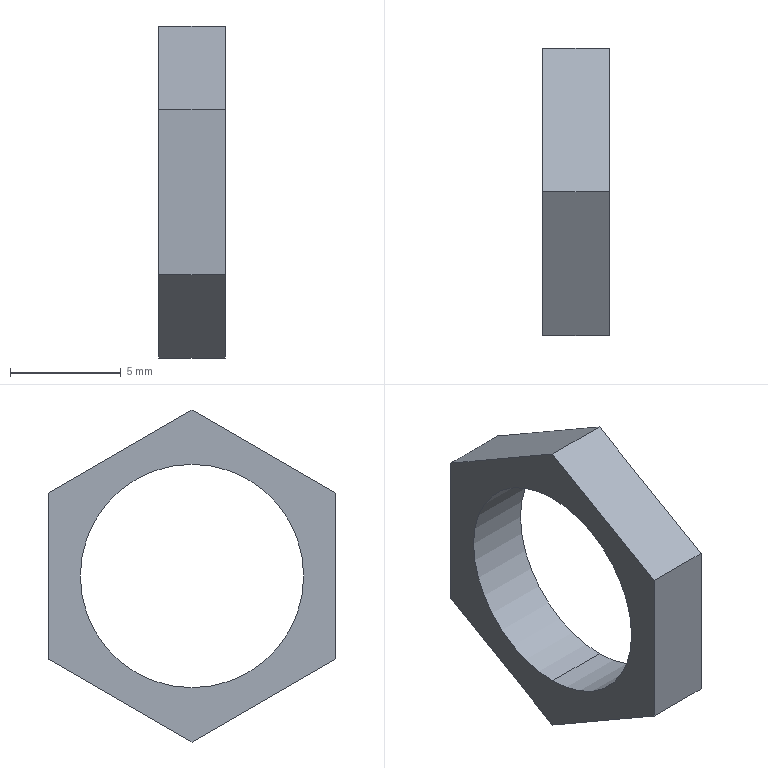Component | SolidWorks | GuideMechanism-1_SwingArm-1_AngleDisplacementSensorNut.1-1 | 1 solid | 10 faces | box 3 x 13 x 15.01 mm | volume 199 mm3 | plane 8 | cylinder 2 | commonest cylinder face diameters 10.1 x2
build123d program:
from build123d import *

# Parameters (mm, degrees)
BOSS_EXTRUDE1_DEPTH    = 3
M10X1_0_TAPPED_HOLE1_D = 10.1


with BuildPart() as part:
    # Sketch1 → Boss-Extrude1 (new body)
    with BuildSketch(Plane.XY):
        Polygon((7.506, 0), (3.753, 6.5), (-3.753, 6.5), (-7.506, 0), (-3.753, -6.5), (3.753, -6.5), align=None)
    extrude(amount=BOSS_EXTRUDE1_DEPTH)

    # M10x1.0 Tapped Hole1 (through all)
    with Locations(Plane(origin=(0, 0, 0), x_dir=(-1, 0, 0), z_dir=(0, 0, -1))):
        with Locations((0, 0)):
            Hole(M10X1_0_TAPPED_HOLE1_D / 2)


solid = part.part

# Placed as in the assembly
solid = solid.moved(Location((-615.272, -568.766, 1326.45), (0, 90, 0)))
STEP:
#1=CARTESIAN_POINT('',(-24.223,-22.392,52.024));
#2=VERTEX_POINT('',#1);
#3=CARTESIAN_POINT('',(-24.223,-22.392,52.421));
#4=VERTEX_POINT('',#3);
#5=CARTESIAN_POINT('',(-24.223,-22.392,52.222));
#6=DIRECTION('',(1.,-0.,0.));
#7=DIRECTION('',(0.,0.,1.));
#8=AXIS2_PLACEMENT_3D('',#5,#6,#7);
#9=CIRCLE('',#8,0.1988);
#10=EDGE_CURVE('',#2,#4,#9,.T.);
#11=ORIENTED_EDGE('',*,*,#10,.F.);
#12=CARTESIAN_POINT('',(-24.105,-22.392,52.024));
#13=VERTEX_POINT('',#12);
#14=CARTESIAN_POINT('',(-24.105,-22.392,52.024));
#15=DIRECTION('',(1.,-0.,0.));
#16=VECTOR('',#15,39.37);
#17=LINE('',#14,#16);
#18=EDGE_CURVE('',#2,#13,#17,.T.);
#19=ORIENTED_EDGE('',*,*,#18,.T.);
#20=CARTESIAN_POINT('',(-24.105,-22.392,52.421));
#21=VERTEX_POINT('',#20);
#22=CARTESIAN_POINT('',(-24.105,-22.392,52.222));
#23=DIRECTION('',(1.,-0.,0.));
#24=DIRECTION('',(0.,0.,1.));
#25=AXIS2_PLACEMENT_3D('',#22,#23,#24);
#26=CIRCLE('',#25,0.1988);
#27=EDGE_CURVE('',#13,#21,#26,.T.);
#28=ORIENTED_EDGE('',*,*,#27,.T.);
#29=CARTESIAN_POINT('',(-24.105,-22.392,52.421));
#30=DIRECTION('',(1.,-0.,0.));
#31=VECTOR('',#30,39.37);
#32=LINE('',#29,#31);
#33=EDGE_CURVE('',#4,#21,#32,.T.);
#34=ORIENTED_EDGE('',*,*,#33,.F.);
#35=EDGE_LOOP('',(#11,#19,#28,#34));
#36=FACE_OUTER_BOUND('',#35,.T.);
#37=CARTESIAN_POINT('',(-24.105,-22.392,52.222));
#38=DIRECTION('',(1.,-0.,0.));
#39=DIRECTION('',(0.,0.,1.));
#40=AXIS2_PLACEMENT_3D('',#37,#38,#39);
#41=CYLINDRICAL_SURFACE('',#40,0.1988);
#42=ADVANCED_FACE('',(#36),#41,.F.);
#43=CARTESIAN_POINT('',(-24.105,-22.136,52.075));
#44=VERTEX_POINT('',#43);
#45=CARTESIAN_POINT('',(-24.105,-22.392,51.927));
#46=VERTEX_POINT('',#45);
#47=CARTESIAN_POINT('',(-24.105,-22.136,52.075));
#48=DIRECTION('',(0.,-0.866,-0.5));
#49=VECTOR('',#48,39.37);
#50=LINE('',#47,#49);
#51=EDGE_CURVE('',#44,#46,#50,.T.);
#52=ORIENTED_EDGE('',*,*,#51,.T.);
#53=CARTESIAN_POINT('',(-24.223,-22.392,51.927));
#54=VERTEX_POINT('',#53);
#55=CARTESIAN_POINT('',(-24.223,-22.392,51.927));
#56=DIRECTION('',(1.,-0.,0.));
#57=VECTOR('',#56,39.37);
#58=LINE('',#55,#57);
#59=EDGE_CURVE('',#54,#46,#58,.T.);
#60=ORIENTED_EDGE('',*,*,#59,.F.);
#61=CARTESIAN_POINT('',(-24.223,-22.136,52.075));
#62=VERTEX_POINT('',#61);
#63=CARTESIAN_POINT('',(-24.223,-22.136,52.075));
#64=DIRECTION('',(0.,-0.866,-0.5));
#65=VECTOR('',#64,39.37);
#66=LINE('',#63,#65);
#67=EDGE_CURVE('',#62,#54,#66,.T.);
#68=ORIENTED_EDGE('',*,*,#67,.F.);
#69=CARTESIAN_POINT('',(-24.223,-22.136,52.075));
#70=DIRECTION('',(1.,-0.,0.));
#71=VECTOR('',#70,39.37);
#72=LINE('',#69,#71);
#73=EDGE_CURVE('',#62,#44,#72,.T.);
#74=ORIENTED_EDGE('',*,*,#73,.T.);
#75=EDGE_LOOP('',(#52,#60,#68,#74));
#76=FACE_OUTER_BOUND('',#75,.T.);
#77=CARTESIAN_POINT('',(-24.223,-22.136,52.075));
#78=DIRECTION('',(-0.,-0.5,0.866));
#79=DIRECTION('',(-0.,0.866,0.5));
#80=AXIS2_PLACEMENT_3D('',#77,#78,#79);
#81=PLANE('',#80);
#82=ADVANCED_FACE('',(#76),#81,.F.);
#83=CARTESIAN_POINT('',(-24.105,-22.648,52.075));
#84=VERTEX_POINT('',#83);
#85=CARTESIAN_POINT('',(-24.105,-22.392,51.927));
#86=DIRECTION('',(-0.,-0.866,0.5));
#87=VECTOR('',#86,39.37);
#88=LINE('',#85,#87);
#89=EDGE_CURVE('',#46,#84,#88,.T.);
#90=ORIENTED_EDGE('',*,*,#89,.T.);
#91=CARTESIAN_POINT('',(-24.223,-22.648,52.075));
#92=VERTEX_POINT('',#91);
#93=CARTESIAN_POINT('',(-24.223,-22.648,52.075));
#94=DIRECTION('',(1.,-0.,0.));
#95=VECTOR('',#94,39.37);
#96=LINE('',#93,#95);
#97=EDGE_CURVE('',#92,#84,#96,.T.);
#98=ORIENTED_EDGE('',*,*,#97,.F.);
#99=CARTESIAN_POINT('',(-24.223,-22.392,51.927));
#100=DIRECTION('',(-0.,-0.866,0.5));
#101=VECTOR('',#100,39.37);
#102=LINE('',#99,#101);
#103=EDGE_CURVE('',#54,#92,#102,.T.);
#104=ORIENTED_EDGE('',*,*,#103,.F.);
#105=ORIENTED_EDGE('',*,*,#59,.T.);
#106=EDGE_LOOP('',(#90,#98,#104,#105));
#107=FACE_OUTER_BOUND('',#106,.T.);
#108=CARTESIAN_POINT('',(-24.223,-22.392,51.927));
#109=DIRECTION('',(-0.,0.5,0.866));
#110=DIRECTION('',(0.,0.866,-0.5));
#111=AXIS2_PLACEMENT_3D('',#108,#109,#110);
#112=PLANE('',#111);
#113=ADVANCED_FACE('',(#107),#112,.F.);
#114=CARTESIAN_POINT('',(-24.105,-22.648,52.37));
#115=VERTEX_POINT('',#114);
#116=CARTESIAN_POINT('',(-24.105,-22.648,52.075));
#117=DIRECTION('',(-0.,0.,1.));
#118=VECTOR('',#117,39.37);
#119=LINE('',#116,#118);
#120=EDGE_CURVE('',#84,#115,#119,.T.);
#121=ORIENTED_EDGE('',*,*,#120,.T.);
#122=CARTESIAN_POINT('',(-24.223,-22.648,52.37));
#123=VERTEX_POINT('',#122);
#124=CARTESIAN_POINT('',(-24.223,-22.648,52.37));
#125=DIRECTION('',(1.,-0.,0.));
#126=VECTOR('',#125,39.37);
#127=LINE('',#124,#126);
#128=EDGE_CURVE('',#123,#115,#127,.T.);
#129=ORIENTED_EDGE('',*,*,#128,.F.);
#130=CARTESIAN_POINT('',(-24.223,-22.648,52.075));
#131=DIRECTION('',(-0.,0.,1.));
#132=VECTOR('',#131,39.37);
#133=LINE('',#130,#132);
#134=EDGE_CURVE('',#92,#123,#133,.T.);
#135=ORIENTED_EDGE('',*,*,#134,.F.);
#136=ORIENTED_EDGE('',*,*,#97,.T.);
#137=EDGE_LOOP('',(#121,#129,#135,#136));
#138=FACE_OUTER_BOUND('',#137,.T.);
#139=CARTESIAN_POINT('',(-24.223,-22.648,52.075));
#140=DIRECTION('',(0.,1.,-0.));
#141=DIRECTION('',(0.,-0.,-1.));
#142=AXIS2_PLACEMENT_3D('',#139,#140,#141);
#143=PLANE('',#142);
#144=ADVANCED_FACE('',(#138),#143,.F.);
#145=CARTESIAN_POINT('',(-24.105,-22.392,52.518));
#146=VERTEX_POINT('',#145);
#147=CARTESIAN_POINT('',(-24.105,-22.648,52.37));
#148=DIRECTION('',(-0.,0.866,0.5));
#149=VECTOR('',#148,39.37);
#150=LINE('',#147,#149);
#151=EDGE_CURVE('',#115,#146,#150,.T.);
#152=ORIENTED_EDGE('',*,*,#151,.T.);
#153=CARTESIAN_POINT('',(-24.223,-22.392,52.518));
#154=VERTEX_POINT('',#153);
#155=CARTESIAN_POINT('',(-24.223,-22.392,52.518));
#156=DIRECTION('',(1.,-0.,0.));
#157=VECTOR('',#156,39.37);
#158=LINE('',#155,#157);
#159=EDGE_CURVE('',#154,#146,#158,.T.);
#160=ORIENTED_EDGE('',*,*,#159,.F.);
#161=CARTESIAN_POINT('',(-24.223,-22.648,52.37));
#162=DIRECTION('',(-0.,0.866,0.5));
#163=VECTOR('',#162,39.37);
#164=LINE('',#161,#163);
#165=EDGE_CURVE('',#123,#154,#164,.T.);
#166=ORIENTED_EDGE('',*,*,#165,.F.);
#167=ORIENTED_EDGE('',*,*,#128,.T.);
#168=EDGE_LOOP('',(#152,#160,#166,#167));
#169=FACE_OUTER_BOUND('',#168,.T.);
#170=CARTESIAN_POINT('',(-24.223,-22.648,52.37));
#171=DIRECTION('',(0.,0.5,-0.866));
#172=DIRECTION('',(0.,-0.866,-0.5));
#173=AXIS2_PLACEMENT_3D('',#170,#171,#172);
#174=PLANE('',#173);
#175=ADVANCED_FACE('',(#169),#174,.F.);
#176=CARTESIAN_POINT('',(-24.105,-22.136,52.37));
#177=VERTEX_POINT('',#176);
#178=CARTESIAN_POINT('',(-24.105,-22.392,52.518));
#179=DIRECTION('',(0.,0.866,-0.5));
#180=VECTOR('',#179,39.37);
#181=LINE('',#178,#180);
#182=EDGE_CURVE('',#146,#177,#181,.T.);
#183=ORIENTED_EDGE('',*,*,#182,.T.);
#184=CARTESIAN_POINT('',(-24.223,-22.136,52.37));
#185=VERTEX_POINT('',#184);
#186=CARTESIAN_POINT('',(-24.223,-22.136,52.37));
#187=DIRECTION('',(1.,-0.,0.));
#188=VECTOR('',#187,39.37);
#189=LINE('',#186,#188);
#190=EDGE_CURVE('',#185,#177,#189,.T.);
#191=ORIENTED_EDGE('',*,*,#190,.F.);
#192=CARTESIAN_POINT('',(-24.223,-22.392,52.518));
#193=DIRECTION('',(0.,0.866,-0.5));
#194=VECTOR('',#193,39.37);
#195=LINE('',#192,#194);
#196=EDGE_CURVE('',#154,#185,#195,.T.);
#197=ORIENTED_EDGE('',*,*,#196,.F.);
#198=ORIENTED_EDGE('',*,*,#159,.T.);
#199=EDGE_LOOP('',(#183,#191,#197,#198));
#200=FACE_OUTER_BOUND('',#199,.T.);
#201=CARTESIAN_POINT('',(-24.223,-22.392,52.518));
#202=DIRECTION('',(0.,-0.5,-0.866));
#203=DIRECTION('',(-0.,-0.866,0.5));
#204=AXIS2_PLACEMENT_3D('',#201,#202,#203);
#205=PLANE('',#204);
#206=ADVANCED_FACE('',(#200),#205,.F.);
#207=CARTESIAN_POINT('',(-24.105,-22.136,52.37));
#208=DIRECTION('',(0.,-0.,-1.));
#209=VECTOR('',#208,39.37);
#210=LINE('',#207,#209);
#211=EDGE_CURVE('',#177,#44,#210,.T.);
#212=ORIENTED_EDGE('',*,*,#211,.T.);
#213=ORIENTED_EDGE('',*,*,#73,.F.);
#214=CARTESIAN_POINT('',(-24.223,-22.136,52.37));
#215=DIRECTION('',(0.,-0.,-1.));
#216=VECTOR('',#215,39.37);
#217=LINE('',#214,#216);
#218=EDGE_CURVE('',#185,#62,#217,.T.);
#219=ORIENTED_EDGE('',*,*,#218,.F.);
#220=ORIENTED_EDGE('',*,*,#190,.T.);
#221=EDGE_LOOP('',(#212,#213,#219,#220));
#222=FACE_OUTER_BOUND('',#221,.T.);
#223=CARTESIAN_POINT('',(-24.223,-22.136,52.37));
#224=DIRECTION('',(-0.,-1.,0.));
#225=DIRECTION('',(-0.,0.,1.));
#226=AXIS2_PLACEMENT_3D('',#223,#224,#225);
#227=PLANE('',#226);
#228=ADVANCED_FACE('',(#222),#227,.F.);
#229=CARTESIAN_POINT('',(-24.223,-22.392,52.222));
#230=DIRECTION('',(1.,-0.,0.));
#231=DIRECTION('',(0.,0.,1.));
#232=AXIS2_PLACEMENT_3D('',#229,#230,#231);
#233=CIRCLE('',#232,0.1988);
#234=EDGE_CURVE('',#4,#2,#233,.T.);
#235=ORIENTED_EDGE('',*,*,#234,.T.);
#236=ORIENTED_EDGE('',*,*,#10,.T.);
#237=EDGE_LOOP('',(#235,#236));
#238=FACE_BOUND('',#237,.T.);
#239=ORIENTED_EDGE('',*,*,#67,.T.);
#240=ORIENTED_EDGE('',*,*,#103,.T.);
#241=ORIENTED_EDGE('',*,*,#134,.T.);
#242=ORIENTED_EDGE('',*,*,#165,.T.);
#243=ORIENTED_EDGE('',*,*,#196,.T.);
#244=ORIENTED_EDGE('',*,*,#218,.T.);
#245=EDGE_LOOP('',(#239,#240,#241,#242,#243,#244));
#246=FACE_OUTER_BOUND('',#245,.T.);
#247=CARTESIAN_POINT('',(-24.223,-22.392,52.222));
#248=DIRECTION('',(-1.,0.,-0.));
#249=DIRECTION('',(0.,0.,-1.));
#250=AXIS2_PLACEMENT_3D('',#247,#248,#249);
#251=PLANE('',#250);
#252=ADVANCED_FACE('',(#238,#246),#251,.T.);
#253=CARTESIAN_POINT('',(-24.105,-22.392,52.222));
#254=DIRECTION('',(1.,-0.,0.));
#255=DIRECTION('',(0.,0.,1.));
#256=AXIS2_PLACEMENT_3D('',#253,#254,#255);
#257=CIRCLE('',#256,0.1988);
#258=EDGE_CURVE('',#21,#13,#257,.T.);
#259=ORIENTED_EDGE('',*,*,#258,.F.);
#260=ORIENTED_EDGE('',*,*,#27,.F.);
#261=EDGE_LOOP('',(#259,#260));
#262=FACE_BOUND('',#261,.T.);
#263=ORIENTED_EDGE('',*,*,#51,.F.);
#264=ORIENTED_EDGE('',*,*,#211,.F.);
#265=ORIENTED_EDGE('',*,*,#182,.F.);
#266=ORIENTED_EDGE('',*,*,#151,.F.);
#267=ORIENTED_EDGE('',*,*,#120,.F.);
#268=ORIENTED_EDGE('',*,*,#89,.F.);
#269=EDGE_LOOP('',(#263,#264,#265,#266,#267,#268));
#270=FACE_OUTER_BOUND('',#269,.T.);
#271=CARTESIAN_POINT('',(-24.105,-22.392,52.222));
#272=DIRECTION('',(-1.,0.,-0.));
#273=DIRECTION('',(0.,0.,-1.));
#274=AXIS2_PLACEMENT_3D('',#271,#272,#273);
#275=PLANE('',#274);
#276=ADVANCED_FACE('',(#262,#270),#275,.F.);
#277=ORIENTED_EDGE('',*,*,#18,.F.);
#278=ORIENTED_EDGE('',*,*,#234,.F.);
#279=ORIENTED_EDGE('',*,*,#33,.T.);
#280=ORIENTED_EDGE('',*,*,#258,.T.);
#281=EDGE_LOOP('',(#277,#278,#279,#280));
#282=FACE_OUTER_BOUND('',#281,.T.);
#283=CARTESIAN_POINT('',(-24.105,-22.392,52.222));
#284=DIRECTION('',(1.,-0.,0.));
#285=DIRECTION('',(0.,0.,1.));
#286=AXIS2_PLACEMENT_3D('',#283,#284,#285);
#287=CYLINDRICAL_SURFACE('',#286,0.1988);
#288=ADVANCED_FACE('',(#282),#287,.F.);
#289=CLOSED_SHELL('',(#42,#82,#113,#144,#175,#206,#228,#252,#276,#288));
#290=MANIFOLD_SOLID_BREP('',#289);
#291=CARTESIAN_POINT('',(0.,0.,0.));
#292=DIRECTION('',(0.,0.,1.));
#293=DIRECTION('',(1.,0.,0.));
#294=AXIS2_PLACEMENT_3D('',#291,#292,#293);
#295=(LENGTH_UNIT()NAMED_UNIT(*)SI_UNIT($,.METRE.));
#296=LENGTH_MEASURE_WITH_UNIT(LENGTH_MEASURE(0.0254),#295);
#297=DIMENSIONAL_EXPONENTS(1.,0.,0.,0.,0.,0.,0.);
#298=(CONVERSION_BASED_UNIT('',#296)LENGTH_UNIT()NAMED_UNIT(#297));
#299=UNCERTAINTY_MEASURE_WITH_UNIT(LENGTH_MEASURE(0.00001),#298,'','');
#300=(NAMED_UNIT(*)PLANE_ANGLE_UNIT()SI_UNIT($,.RADIAN.));
#301=(NAMED_UNIT(*)SI_UNIT($,.STERADIAN.)SOLID_ANGLE_UNIT());
#302=(GEOMETRIC_REPRESENTATION_CONTEXT(3)GLOBAL_UNCERTAINTY_ASSIGNED_CONTEXT((#299))GLOBAL_UNIT_ASSIGNED_CONTEXT((#298,#300,#301))REPRESENTATION_CONTEXT('',''));
#303=ADVANCED_BREP_SHAPE_REPRESENTATION('',(#290,#294),#302);
#304=COLOUR_RGB('',0.7922,0.8196,0.9333);
#305=FILL_AREA_STYLE_COLOUR('',#304);
#306=FILL_AREA_STYLE('',(#305));
#307=SURFACE_STYLE_FILL_AREA(#306);
#308=SURFACE_SIDE_STYLE('',(#307));
#309=SURFACE_STYLE_USAGE(.BOTH.,#308);
#310=PRESENTATION_STYLE_ASSIGNMENT((#309));
#311=STYLED_ITEM('',(#310),#290);
#312=(LENGTH_UNIT()NAMED_UNIT(*)SI_UNIT($,.METRE.));
#313=LENGTH_MEASURE_WITH_UNIT(LENGTH_MEASURE(0.0254),#312);
#314=DIMENSIONAL_EXPONENTS(1.,0.,0.,0.,0.,0.,0.);
#315=(CONVERSION_BASED_UNIT('',#313)LENGTH_UNIT()NAMED_UNIT(#314));
#316=UNCERTAINTY_MEASURE_WITH_UNIT(LENGTH_MEASURE(0.00001),#315,'','');
#317=(NAMED_UNIT(*)PLANE_ANGLE_UNIT()SI_UNIT($,.RADIAN.));
#318=(NAMED_UNIT(*)SI_UNIT($,.STERADIAN.)SOLID_ANGLE_UNIT());
#319=(GEOMETRIC_REPRESENTATION_CONTEXT(3)GLOBAL_UNCERTAINTY_ASSIGNED_CONTEXT((#316))GLOBAL_UNIT_ASSIGNED_CONTEXT((#315,#317,#318))REPRESENTATION_CONTEXT('',''));
#320=MECHANICAL_DESIGN_GEOMETRIC_PRESENTATION_REPRESENTATION('',(#311),#319);
#321=PRESENTATION_LAYER_ASSIGNMENT('','',(#311));